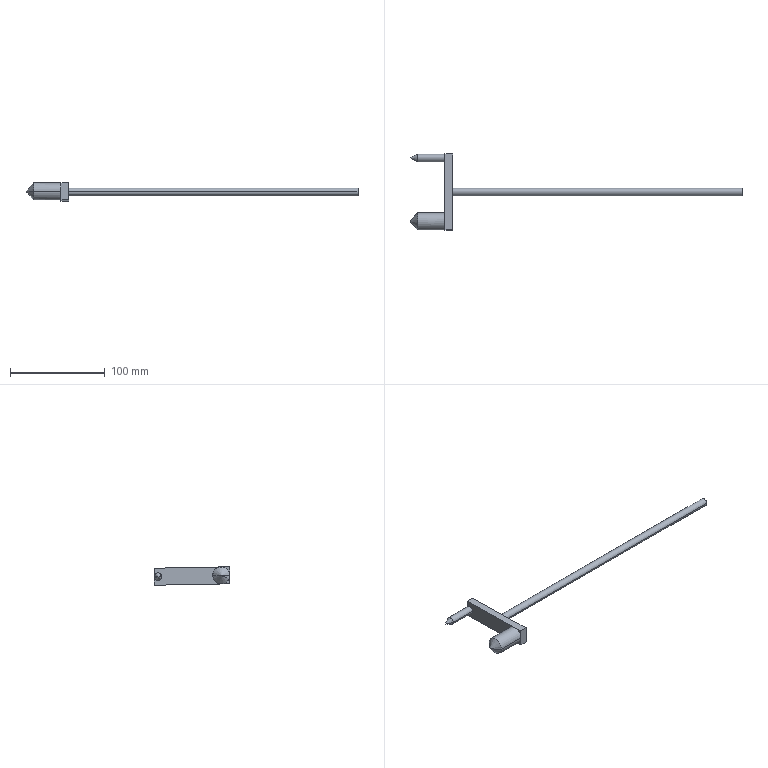Component | SolidWorks | RockerArm-1 | 1 solid | 19 faces | box 351 x 80.32 x 19.49 mm | volume 36551 mm3 | plane 9 | cylinder 6 | cone 4 | commonest cylinder face diameters 8 x4 18 x2
build123d program:
from build123d import *

# Parameters (mm, degrees)
SKETCH1_R           = 4
BOSS_EXTRUDE1_DEPTH = 306
SKETCH2_W           = 80
SKETCH2_H           = 18
BOSS_EXTRUDE2_DEPTH = 8
SKETCH4_R           = 9
SKETCH4_R_2         = 4
BOSS_EXTRUDE3_DEPTH = 37
CUT_EXTRUDE1_START  = -8
SKETCH6_R           = 9
CUT_EXTRUDE1_DEPTH  = 8
CUT_EXTRUDE2_START  = -8
SKETCH7_R           = 4
CUT_EXTRUDE2_DEPTH  = 8


with BuildPart() as part:
    # Sketch1 → Boss-Extrude1 (new body)
    with BuildSketch(Plane(origin=(0, 0, 0), x_dir=(0, 0, -1), z_dir=(1, 0, 0))):
        Circle(SKETCH1_R)
    extrude(amount=BOSS_EXTRUDE1_DEPTH)

    # Sketch2 → Boss-Extrude2 (add)
    with BuildSketch(Plane(origin=(306, 0, 0), x_dir=(0, 0, -1), z_dir=(1, 0, 0))):
        Rectangle(SKETCH2_W, SKETCH2_H)
    extrude(amount=BOSS_EXTRUDE2_DEPTH)

    # Sketch4 → Boss-Extrude3 (add)
    with BuildSketch(Plane(origin=(314, 0, 0), x_dir=(0, 0, -1), z_dir=(1, 0, 0))):
        with Locations(Location((-31, 0, 0), (0, 0, 180))):
            Circle(SKETCH4_R)
        with Locations((36, 0)):
            Circle(SKETCH4_R_2)
    extrude(amount=BOSS_EXTRUDE3_DEPTH)

    # Sketch6 → Cut-Extrude1 (cut)
    with BuildSketch(Plane(origin=(351, 0, 0), x_dir=(0, 0, -1), z_dir=(1, 0, 0)).offset(CUT_EXTRUDE1_START)):
        with Locations(Location((-31, 0, 0), (0, 0, 180))):
            Circle(SKETCH6_R)
    extrude(amount=CUT_EXTRUDE1_DEPTH, mode=Mode.SUBTRACT)

    # Sketch5 → Revolve1 (revolve)
    with BuildSketch(Plane(origin=(0, 0, 0), x_dir=(1, 0, 0), z_dir=(0, 1, 0)), mode=Mode.PRIVATE) as revolve1_sk:
        Polygon((351, -31), (343, -31), (343, -22), align=None)
    revolve(revolve1_sk.sketch.rotate(Axis((351, 0, 31), (-1, 0, 0)), 180), axis=Axis((351, 0, 31), (-1, 0, 0)))

    # Sketch7 → Cut-Extrude2 (cut)
    with BuildSketch(Plane(origin=(351, 0, 0), x_dir=(0, 0, -1), z_dir=(1, 0, 0)).offset(CUT_EXTRUDE2_START)):
        with Locations((36, 0)):
            Circle(SKETCH7_R)
    extrude(amount=CUT_EXTRUDE2_DEPTH, mode=Mode.SUBTRACT)

    # Sketch8 → Revolve2 (revolve)
    with BuildSketch(Plane(origin=(0, 0, 0), x_dir=(1, 0, 0), z_dir=(0, 1, 0)), mode=Mode.PRIVATE) as revolve2_sk:
        Polygon((343, 36), (351, 36), (343, 40), align=None)
    revolve(revolve2_sk.sketch.rotate(Axis((343, 0, -36), (1, 0, 0)), 180), axis=Axis((343, 0, -36), (1, 0, 0)))


solid = part.part

# Placed as in the assembly
solid = solid.moved(Location((890.528, 15.81, -277), (88.932, 0, -180)))
STEP:
#1=COLOUR_RGB('',0.7922,0.8196,0.9333);
#2=FILL_AREA_STYLE_COLOUR('',#1);
#3=FILL_AREA_STYLE('',(#2));
#4=SURFACE_STYLE_FILL_AREA(#3);
#5=SURFACE_SIDE_STYLE('',(#4));
#6=SURFACE_STYLE_USAGE(.BOTH.,#5);
#7=PRESENTATION_STYLE_ASSIGNMENT((#6));
#8=CARTESIAN_POINT('',(21.241,2.04,-10.932));
#9=VERTEX_POINT('',#8);
#10=CARTESIAN_POINT('',(21.556,1.882,-10.929));
#11=VERTEX_POINT('',#10);
#12=CARTESIAN_POINT('',(21.241,2.04,-10.932));
#13=DIRECTION('',(0.8944,-0.4471,0.008333));
#14=VECTOR('',#13,39.37);
#15=LINE('',#12,#14);
#16=EDGE_CURVE('',#9,#11,#15,.T.);
#17=ORIENTED_EDGE('',*,*,#16,.F.);
#18=CARTESIAN_POINT('',(21.556,2.197,-10.935));
#19=VERTEX_POINT('',#18);
#20=CARTESIAN_POINT('',(21.241,2.04,-10.932));
#21=DIRECTION('',(0.8944,0.4471,-0.008333));
#22=VECTOR('',#21,39.37);
#23=LINE('',#20,#22);
#24=EDGE_CURVE('',#9,#19,#23,.T.);
#25=ORIENTED_EDGE('',*,*,#24,.T.);
#26=CARTESIAN_POINT('',(21.556,2.04,-10.932));
#27=DIRECTION('',(-1.,-0.,-0.));
#28=DIRECTION('',(0.,0.9998,-0.01863));
#29=AXIS2_PLACEMENT_3D('',#26,#27,#28);
#30=CIRCLE('',#29,0.1575);
#31=EDGE_CURVE('',#19,#11,#30,.T.);
#32=ORIENTED_EDGE('',*,*,#31,.T.);
#33=EDGE_LOOP('',(#17,#25,#32));
#34=FACE_OUTER_BOUND('',#33,.T.);
#35=CARTESIAN_POINT('',(60.611,2.04,-10.932));
#36=DIRECTION('',(1.,0.,0.));
#37=DIRECTION('',(0.,-0.9998,0.01863));
#38=AXIS2_PLACEMENT_3D('',#35,#36,#37);
#39=CONICAL_SURFACE('',#38,19.685,0.4636);
#40=ADVANCED_FACE('',(#34),#39,.T.);
#41=CARTESIAN_POINT('',(21.241,-0.5978,-10.883));
#42=VERTEX_POINT('',#41);
#43=CARTESIAN_POINT('',(21.556,-0.9521,-10.876));
#44=VERTEX_POINT('',#43);
#45=CARTESIAN_POINT('',(21.241,-0.5978,-10.883));
#46=DIRECTION('',(0.6644,-0.7473,0.01393));
#47=VECTOR('',#46,39.37);
#48=LINE('',#45,#47);
#49=EDGE_CURVE('',#42,#44,#48,.T.);
#50=ORIENTED_EDGE('',*,*,#49,.F.);
#51=CARTESIAN_POINT('',(21.556,-0.2435,-10.889));
#52=VERTEX_POINT('',#51);
#53=CARTESIAN_POINT('',(21.241,-0.5978,-10.883));
#54=DIRECTION('',(0.6644,0.7473,-0.01393));
#55=VECTOR('',#54,39.37);
#56=LINE('',#53,#55);
#57=EDGE_CURVE('',#42,#52,#56,.T.);
#58=ORIENTED_EDGE('',*,*,#57,.T.);
#59=CARTESIAN_POINT('',(21.556,-0.5978,-10.883));
#60=DIRECTION('',(-1.,-0.,-0.));
#61=DIRECTION('',(0.,0.9998,-0.01863));
#62=AXIS2_PLACEMENT_3D('',#59,#60,#61);
#63=CIRCLE('',#62,0.3543);
#64=EDGE_CURVE('',#52,#44,#63,.T.);
#65=ORIENTED_EDGE('',*,*,#64,.T.);
#66=EDGE_LOOP('',(#50,#58,#65));
#67=FACE_OUTER_BOUND('',#66,.T.);
#68=CARTESIAN_POINT('',(60.611,-0.5978,-10.883));
#69=DIRECTION('',(1.,0.,0.));
#70=DIRECTION('',(0.,-0.9998,0.01863));
#71=AXIS2_PLACEMENT_3D('',#68,#69,#70);
#72=CONICAL_SURFACE('',#71,44.291,0.8442);
#73=ADVANCED_FACE('',(#67),#72,.T.);
#74=CARTESIAN_POINT('',(23.013,0.7799,-10.908));
#75=VERTEX_POINT('',#74);
#76=CARTESIAN_POINT('',(23.013,0.465,-10.903));
#77=VERTEX_POINT('',#76);
#78=CARTESIAN_POINT('',(23.013,0.6225,-10.906));
#79=DIRECTION('',(-1.,-0.,-0.));
#80=DIRECTION('',(0.,0.9998,-0.01863));
#81=AXIS2_PLACEMENT_3D('',#78,#79,#80);
#82=CIRCLE('',#81,0.1575);
#83=EDGE_CURVE('',#75,#77,#82,.T.);
#84=ORIENTED_EDGE('',*,*,#83,.F.);
#85=CARTESIAN_POINT('',(35.06,0.7799,-10.908));
#86=VERTEX_POINT('',#85);
#87=CARTESIAN_POINT('',(23.013,0.7799,-10.908));
#88=DIRECTION('',(1.,0.,0.));
#89=VECTOR('',#88,39.37);
#90=LINE('',#87,#89);
#91=EDGE_CURVE('',#75,#86,#90,.T.);
#92=ORIENTED_EDGE('',*,*,#91,.T.);
#93=CARTESIAN_POINT('',(35.06,0.465,-10.903));
#94=VERTEX_POINT('',#93);
#95=CARTESIAN_POINT('',(35.06,0.6225,-10.906));
#96=DIRECTION('',(-1.,-0.,-0.));
#97=DIRECTION('',(0.,0.9998,-0.01863));
#98=AXIS2_PLACEMENT_3D('',#95,#96,#97);
#99=CIRCLE('',#98,0.1575);
#100=EDGE_CURVE('',#86,#94,#99,.T.);
#101=ORIENTED_EDGE('',*,*,#100,.T.);
#102=CARTESIAN_POINT('',(23.013,0.465,-10.903));
#103=DIRECTION('',(1.,0.,0.));
#104=VECTOR('',#103,39.37);
#105=LINE('',#102,#104);
#106=EDGE_CURVE('',#77,#94,#105,.T.);
#107=ORIENTED_EDGE('',*,*,#106,.F.);
#108=EDGE_LOOP('',(#84,#92,#101,#107));
#109=FACE_OUTER_BOUND('',#108,.T.);
#110=CARTESIAN_POINT('',(23.013,0.6225,-10.906));
#111=DIRECTION('',(1.,0.,0.));
#112=DIRECTION('',(0.,-0.9998,0.01863));
#113=AXIS2_PLACEMENT_3D('',#110,#111,#112);
#114=CYLINDRICAL_SURFACE('',#113,0.1575);
#115=ADVANCED_FACE('',(#109),#114,.T.);
#116=ORIENTED_EDGE('',*,*,#64,.F.);
#117=CARTESIAN_POINT('',(22.698,-0.2435,-10.889));
#118=VERTEX_POINT('',#117);
#119=CARTESIAN_POINT('',(21.241,-0.2435,-10.889));
#120=DIRECTION('',(1.,0.,0.));
#121=VECTOR('',#120,39.37);
#122=LINE('',#119,#121);
#123=EDGE_CURVE('',#52,#118,#122,.T.);
#124=ORIENTED_EDGE('',*,*,#123,.T.);
#125=CARTESIAN_POINT('',(22.698,-0.6044,-11.237));
#126=VERTEX_POINT('',#125);
#127=CARTESIAN_POINT('',(22.698,-0.5978,-10.883));
#128=DIRECTION('',(-1.,-0.,-0.));
#129=DIRECTION('',(0.,0.9998,-0.01863));
#130=AXIS2_PLACEMENT_3D('',#127,#128,#129);
#131=CIRCLE('',#130,0.3543);
#132=EDGE_CURVE('',#118,#126,#131,.T.);
#133=ORIENTED_EDGE('',*,*,#132,.T.);
#134=CARTESIAN_POINT('',(22.698,-0.9521,-10.876));
#135=VERTEX_POINT('',#134);
#136=CARTESIAN_POINT('',(22.698,-0.5978,-10.883));
#137=DIRECTION('',(-1.,-0.,-0.));
#138=DIRECTION('',(0.,0.9998,-0.01863));
#139=AXIS2_PLACEMENT_3D('',#136,#137,#138);
#140=CIRCLE('',#139,0.3543);
#141=EDGE_CURVE('',#126,#135,#140,.T.);
#142=ORIENTED_EDGE('',*,*,#141,.T.);
#143=CARTESIAN_POINT('',(21.241,-0.9521,-10.876));
#144=DIRECTION('',(1.,0.,0.));
#145=VECTOR('',#144,39.37);
#146=LINE('',#143,#145);
#147=EDGE_CURVE('',#44,#135,#146,.T.);
#148=ORIENTED_EDGE('',*,*,#147,.F.);
#149=EDGE_LOOP('',(#116,#124,#133,#142,#148));
#150=FACE_OUTER_BOUND('',#149,.T.);
#151=CARTESIAN_POINT('',(21.241,-0.5978,-10.883));
#152=DIRECTION('',(1.,0.,0.));
#153=DIRECTION('',(0.,-0.9998,0.01863));
#154=AXIS2_PLACEMENT_3D('',#151,#152,#153);
#155=CYLINDRICAL_SURFACE('',#154,0.3543);
#156=ADVANCED_FACE('',(#150),#155,.T.);
#157=ORIENTED_EDGE('',*,*,#31,.F.);
#158=CARTESIAN_POINT('',(22.698,2.197,-10.935));
#159=VERTEX_POINT('',#158);
#160=CARTESIAN_POINT('',(21.241,2.197,-10.935));
#161=DIRECTION('',(1.,0.,0.));
#162=VECTOR('',#161,39.37);
#163=LINE('',#160,#162);
#164=EDGE_CURVE('',#19,#159,#163,.T.);
#165=ORIENTED_EDGE('',*,*,#164,.T.);
#166=CARTESIAN_POINT('',(22.698,1.882,-10.929));
#167=VERTEX_POINT('',#166);
#168=CARTESIAN_POINT('',(22.698,2.04,-10.932));
#169=DIRECTION('',(-1.,-0.,-0.));
#170=DIRECTION('',(0.,0.9998,-0.01863));
#171=AXIS2_PLACEMENT_3D('',#168,#169,#170);
#172=CIRCLE('',#171,0.1575);
#173=EDGE_CURVE('',#159,#167,#172,.T.);
#174=ORIENTED_EDGE('',*,*,#173,.T.);
#175=CARTESIAN_POINT('',(21.241,1.882,-10.929));
#176=DIRECTION('',(1.,0.,0.));
#177=VECTOR('',#176,39.37);
#178=LINE('',#175,#177);
#179=EDGE_CURVE('',#11,#167,#178,.T.);
#180=ORIENTED_EDGE('',*,*,#179,.F.);
#181=EDGE_LOOP('',(#157,#165,#174,#180));
#182=FACE_OUTER_BOUND('',#181,.T.);
#183=CARTESIAN_POINT('',(21.241,2.04,-10.932));
#184=DIRECTION('',(1.,0.,0.));
#185=DIRECTION('',(0.,-0.9998,0.01863));
#186=AXIS2_PLACEMENT_3D('',#183,#184,#185);
#187=CYLINDRICAL_SURFACE('',#186,0.1575);
#188=ADVANCED_FACE('',(#182),#187,.T.);
#189=ORIENTED_EDGE('',*,*,#164,.F.);
#190=CARTESIAN_POINT('',(21.556,2.04,-10.932));
#191=DIRECTION('',(-1.,-0.,-0.));
#192=DIRECTION('',(0.,0.9998,-0.01863));
#193=AXIS2_PLACEMENT_3D('',#190,#191,#192);
#194=CIRCLE('',#193,0.1575);
#195=EDGE_CURVE('',#11,#19,#194,.T.);
#196=ORIENTED_EDGE('',*,*,#195,.F.);
#197=ORIENTED_EDGE('',*,*,#179,.T.);
#198=CARTESIAN_POINT('',(22.698,2.04,-10.932));
#199=DIRECTION('',(-1.,-0.,-0.));
#200=DIRECTION('',(0.,0.9998,-0.01863));
#201=AXIS2_PLACEMENT_3D('',#198,#199,#200);
#202=CIRCLE('',#201,0.1575);
#203=EDGE_CURVE('',#167,#159,#202,.T.);
#204=ORIENTED_EDGE('',*,*,#203,.T.);
#205=EDGE_LOOP('',(#189,#196,#197,#204));
#206=FACE_OUTER_BOUND('',#205,.T.);
#207=CARTESIAN_POINT('',(21.241,2.04,-10.932));
#208=DIRECTION('',(1.,0.,0.));
#209=DIRECTION('',(0.,-0.9998,0.01863));
#210=AXIS2_PLACEMENT_3D('',#207,#208,#209);
#211=CYLINDRICAL_SURFACE('',#210,0.1575);
#212=ADVANCED_FACE('',(#206),#211,.T.);
#213=ORIENTED_EDGE('',*,*,#123,.F.);
#214=CARTESIAN_POINT('',(21.556,-0.5978,-10.883));
#215=DIRECTION('',(-1.,-0.,-0.));
#216=DIRECTION('',(0.,0.9998,-0.01863));
#217=AXIS2_PLACEMENT_3D('',#214,#215,#216);
#218=CIRCLE('',#217,0.3543);
#219=EDGE_CURVE('',#44,#52,#218,.T.);
#220=ORIENTED_EDGE('',*,*,#219,.F.);
#221=ORIENTED_EDGE('',*,*,#147,.T.);
#222=CARTESIAN_POINT('',(22.698,-0.5912,-10.529));
#223=VERTEX_POINT('',#222);
#224=CARTESIAN_POINT('',(22.698,-0.5978,-10.883));
#225=DIRECTION('',(-1.,-0.,-0.));
#226=DIRECTION('',(0.,0.9998,-0.01863));
#227=AXIS2_PLACEMENT_3D('',#224,#225,#226);
#228=CIRCLE('',#227,0.3543);
#229=EDGE_CURVE('',#135,#223,#228,.T.);
#230=ORIENTED_EDGE('',*,*,#229,.T.);
#231=CARTESIAN_POINT('',(22.698,-0.5978,-10.883));
#232=DIRECTION('',(-1.,-0.,-0.));
#233=DIRECTION('',(0.,0.9998,-0.01863));
#234=AXIS2_PLACEMENT_3D('',#231,#232,#233);
#235=CIRCLE('',#234,0.3543);
#236=EDGE_CURVE('',#223,#118,#235,.T.);
#237=ORIENTED_EDGE('',*,*,#236,.T.);
#238=EDGE_LOOP('',(#213,#220,#221,#230,#237));
#239=FACE_OUTER_BOUND('',#238,.T.);
#240=CARTESIAN_POINT('',(21.241,-0.5978,-10.883));
#241=DIRECTION('',(1.,0.,0.));
#242=DIRECTION('',(0.,-0.9998,0.01863));
#243=AXIS2_PLACEMENT_3D('',#240,#241,#242);
#244=CYLINDRICAL_SURFACE('',#243,0.3543);
#245=ADVANCED_FACE('',(#239),#244,.T.);
#246=CARTESIAN_POINT('',(22.698,2.204,-10.581));
#247=VERTEX_POINT('',#246);
#248=CARTESIAN_POINT('',(22.698,2.19,-11.289));
#249=DIRECTION('',(0.,-0.01863,-0.9998));
#250=VECTOR('',#249,39.37);
#251=LINE('',#248,#250);
#252=EDGE_CURVE('',#247,#159,#251,.T.);
#253=ORIENTED_EDGE('',*,*,#252,.T.);
#254=ORIENTED_EDGE('',*,*,#203,.F.);
#255=ORIENTED_EDGE('',*,*,#173,.F.);
#256=CARTESIAN_POINT('',(22.698,2.19,-11.289));
#257=VERTEX_POINT('',#256);
#258=CARTESIAN_POINT('',(22.698,2.19,-11.289));
#259=DIRECTION('',(0.,-0.01863,-0.9998));
#260=VECTOR('',#259,39.37);
#261=LINE('',#258,#260);
#262=EDGE_CURVE('',#159,#257,#261,.T.);
#263=ORIENTED_EDGE('',*,*,#262,.T.);
#264=CARTESIAN_POINT('',(22.698,2.19,-11.289));
#265=DIRECTION('',(0.,-0.9998,0.01863));
#266=VECTOR('',#265,39.37);
#267=LINE('',#264,#266);
#268=EDGE_CURVE('',#257,#126,#267,.T.);
#269=ORIENTED_EDGE('',*,*,#268,.T.);
#270=ORIENTED_EDGE('',*,*,#132,.F.);
#271=ORIENTED_EDGE('',*,*,#236,.F.);
#272=CARTESIAN_POINT('',(22.698,2.204,-10.581));
#273=DIRECTION('',(-0.,0.9998,-0.01863));
#274=VECTOR('',#273,39.37);
#275=LINE('',#272,#274);
#276=EDGE_CURVE('',#223,#247,#275,.T.);
#277=ORIENTED_EDGE('',*,*,#276,.T.);
#278=EDGE_LOOP('',(#253,#254,#255,#263,#269,#270,#271,#277));
#279=FACE_OUTER_BOUND('',#278,.T.);
#280=CARTESIAN_POINT('',(22.698,0.6225,-10.906));
#281=DIRECTION('',(1.,0.,0.));
#282=DIRECTION('',(0.,-0.9998,0.01863));
#283=AXIS2_PLACEMENT_3D('',#280,#281,#282);
#284=PLANE('',#283);
#285=ADVANCED_FACE('',(#279),#284,.F.);
#286=ORIENTED_EDGE('',*,*,#141,.F.);
#287=CARTESIAN_POINT('',(22.698,-0.9587,-11.23));
#288=VERTEX_POINT('',#287);
#289=CARTESIAN_POINT('',(22.698,2.19,-11.289));
#290=DIRECTION('',(0.,-0.9998,0.01863));
#291=VECTOR('',#290,39.37);
#292=LINE('',#289,#291);
#293=EDGE_CURVE('',#126,#288,#292,.T.);
#294=ORIENTED_EDGE('',*,*,#293,.T.);
#295=CARTESIAN_POINT('',(22.698,-0.9587,-11.23));
#296=DIRECTION('',(-0.,0.01863,0.9998));
#297=VECTOR('',#296,39.37);
#298=LINE('',#295,#297);
#299=EDGE_CURVE('',#288,#135,#298,.T.);
#300=ORIENTED_EDGE('',*,*,#299,.T.);
#301=EDGE_LOOP('',(#286,#294,#300));
#302=FACE_OUTER_BOUND('',#301,.T.);
#303=CARTESIAN_POINT('',(22.698,0.6225,-10.906));
#304=DIRECTION('',(1.,0.,0.));
#305=DIRECTION('',(0.,-0.9998,0.01863));
#306=AXIS2_PLACEMENT_3D('',#303,#304,#305);
#307=PLANE('',#306);
#308=ADVANCED_FACE('',(#302),#307,.F.);
#309=ORIENTED_EDGE('',*,*,#229,.F.);
#310=CARTESIAN_POINT('',(22.698,-0.9455,-10.522));
#311=VERTEX_POINT('',#310);
#312=CARTESIAN_POINT('',(22.698,-0.9587,-11.23));
#313=DIRECTION('',(-0.,0.01863,0.9998));
#314=VECTOR('',#313,39.37);
#315=LINE('',#312,#314);
#316=EDGE_CURVE('',#135,#311,#315,.T.);
#317=ORIENTED_EDGE('',*,*,#316,.T.);
#318=CARTESIAN_POINT('',(22.698,2.204,-10.581));
#319=DIRECTION('',(-0.,0.9998,-0.01863));
#320=VECTOR('',#319,39.37);
#321=LINE('',#318,#320);
#322=EDGE_CURVE('',#311,#223,#321,.T.);
#323=ORIENTED_EDGE('',*,*,#322,.T.);
#324=EDGE_LOOP('',(#309,#317,#323));
#325=FACE_OUTER_BOUND('',#324,.T.);
#326=CARTESIAN_POINT('',(22.698,0.6225,-10.906));
#327=DIRECTION('',(1.,0.,0.));
#328=DIRECTION('',(0.,-0.9998,0.01863));
#329=AXIS2_PLACEMENT_3D('',#326,#327,#328);
#330=PLANE('',#329);
#331=ADVANCED_FACE('',(#325),#330,.F.);
#332=ORIENTED_EDGE('',*,*,#91,.F.);
#333=CARTESIAN_POINT('',(23.013,0.6225,-10.906));
#334=DIRECTION('',(-1.,-0.,-0.));
#335=DIRECTION('',(0.,0.9998,-0.01863));
#336=AXIS2_PLACEMENT_3D('',#333,#334,#335);
#337=CIRCLE('',#336,0.1575);
#338=EDGE_CURVE('',#77,#75,#337,.T.);
#339=ORIENTED_EDGE('',*,*,#338,.F.);
#340=ORIENTED_EDGE('',*,*,#106,.T.);
#341=CARTESIAN_POINT('',(35.06,0.6225,-10.906));
#342=DIRECTION('',(-1.,-0.,-0.));
#343=DIRECTION('',(0.,0.9998,-0.01863));
#344=AXIS2_PLACEMENT_3D('',#341,#342,#343);
#345=CIRCLE('',#344,0.1575);
#346=EDGE_CURVE('',#94,#86,#345,.T.);
#347=ORIENTED_EDGE('',*,*,#346,.T.);
#348=EDGE_LOOP('',(#332,#339,#340,#347));
#349=FACE_OUTER_BOUND('',#348,.T.);
#350=CARTESIAN_POINT('',(23.013,0.6225,-10.906));
#351=DIRECTION('',(1.,0.,0.));
#352=DIRECTION('',(0.,-0.9998,0.01863));
#353=AXIS2_PLACEMENT_3D('',#350,#351,#352);
#354=CYLINDRICAL_SURFACE('',#353,0.1575);
#355=ADVANCED_FACE('',(#349),#354,.T.);
#356=ORIENTED_EDGE('',*,*,#346,.F.);
#357=ORIENTED_EDGE('',*,*,#100,.F.);
#358=EDGE_LOOP('',(#356,#357));
#359=FACE_OUTER_BOUND('',#358,.T.);
#360=CARTESIAN_POINT('',(35.06,0.6225,-10.906));
#361=DIRECTION('',(-1.,-0.,-0.));
#362=DIRECTION('',(-0.,0.9998,-0.01863));
#363=AXIS2_PLACEMENT_3D('',#360,#361,#362);
#364=PLANE('',#363);
#365=ADVANCED_FACE('',(#359),#364,.F.);
#366=CARTESIAN_POINT('',(23.013,-0.9587,-11.23));
#367=VERTEX_POINT('',#366);
#368=CARTESIAN_POINT('',(23.013,-0.9455,-10.522));
#369=VERTEX_POINT('',#368);
#370=CARTESIAN_POINT('',(23.013,-0.9587,-11.23));
#371=DIRECTION('',(-0.,0.01863,0.9998));
#372=VECTOR('',#371,39.37);
#373=LINE('',#370,#372);
#374=EDGE_CURVE('',#367,#369,#373,.T.);
#375=ORIENTED_EDGE('',*,*,#374,.F.);
#376=CARTESIAN_POINT('',(23.013,2.19,-11.289));
#377=VERTEX_POINT('',#376);
#378=CARTESIAN_POINT('',(23.013,2.19,-11.289));
#379=DIRECTION('',(0.,-0.9998,0.01863));
#380=VECTOR('',#379,39.37);
#381=LINE('',#378,#380);
#382=EDGE_CURVE('',#377,#367,#381,.T.);
#383=ORIENTED_EDGE('',*,*,#382,.F.);
#384=CARTESIAN_POINT('',(23.013,2.204,-10.581));
#385=VERTEX_POINT('',#384);
#386=CARTESIAN_POINT('',(23.013,2.19,-11.289));
#387=DIRECTION('',(0.,-0.01863,-0.9998));
#388=VECTOR('',#387,39.37);
#389=LINE('',#386,#388);
#390=EDGE_CURVE('',#385,#377,#389,.T.);
#391=ORIENTED_EDGE('',*,*,#390,.F.);
#392=CARTESIAN_POINT('',(23.013,2.204,-10.581));
#393=DIRECTION('',(-0.,0.9998,-0.01863));
#394=VECTOR('',#393,39.37);
#395=LINE('',#392,#394);
#396=EDGE_CURVE('',#369,#385,#395,.T.);
#397=ORIENTED_EDGE('',*,*,#396,.F.);
#398=EDGE_LOOP('',(#375,#383,#391,#397));
#399=FACE_OUTER_BOUND('',#398,.T.);
#400=ORIENTED_EDGE('',*,*,#338,.T.);
#401=ORIENTED_EDGE('',*,*,#83,.T.);
#402=EDGE_LOOP('',(#400,#401));
#403=FACE_BOUND('',#402,.T.);
#404=CARTESIAN_POINT('',(23.013,0.6225,-10.906));
#405=DIRECTION('',(1.,0.,0.));
#406=DIRECTION('',(0.,-0.9998,0.01863));
#407=AXIS2_PLACEMENT_3D('',#404,#405,#406);
#408=PLANE('',#407);
#409=ADVANCED_FACE('',(#399,#403),#408,.T.);
#410=ORIENTED_EDGE('',*,*,#374,.T.);
#411=CARTESIAN_POINT('',(22.698,-0.9455,-10.522));
#412=DIRECTION('',(1.,0.,0.));
#413=VECTOR('',#412,39.37);
#414=LINE('',#411,#413);
#415=EDGE_CURVE('',#311,#369,#414,.T.);
#416=ORIENTED_EDGE('',*,*,#415,.F.);
#417=ORIENTED_EDGE('',*,*,#316,.F.);
#418=ORIENTED_EDGE('',*,*,#299,.F.);
#419=CARTESIAN_POINT('',(22.698,-0.9587,-11.23));
#420=DIRECTION('',(1.,0.,0.));
#421=VECTOR('',#420,39.37);
#422=LINE('',#419,#421);
#423=EDGE_CURVE('',#288,#367,#422,.T.);
#424=ORIENTED_EDGE('',*,*,#423,.T.);
#425=EDGE_LOOP('',(#410,#416,#417,#418,#424));
#426=FACE_OUTER_BOUND('',#425,.T.);
#427=CARTESIAN_POINT('',(22.698,-0.9587,-11.23));
#428=DIRECTION('',(-0.,0.9998,-0.01863));
#429=DIRECTION('',(1.,0.,0.));
#430=AXIS2_PLACEMENT_3D('',#427,#428,#429);
#431=PLANE('',#430);
#432=ADVANCED_FACE('',(#426),#431,.F.);
#433=ORIENTED_EDGE('',*,*,#396,.T.);
#434=CARTESIAN_POINT('',(22.698,2.204,-10.581));
#435=DIRECTION('',(1.,0.,0.));
#436=VECTOR('',#435,39.37);
#437=LINE('',#434,#436);
#438=EDGE_CURVE('',#247,#385,#437,.T.);
#439=ORIENTED_EDGE('',*,*,#438,.F.);
#440=ORIENTED_EDGE('',*,*,#276,.F.);
#441=ORIENTED_EDGE('',*,*,#322,.F.);
#442=ORIENTED_EDGE('',*,*,#415,.T.);
#443=EDGE_LOOP('',(#433,#439,#440,#441,#442));
#444=FACE_OUTER_BOUND('',#443,.T.);
#445=CARTESIAN_POINT('',(22.698,2.204,-10.581));
#446=DIRECTION('',(0.,-0.01863,-0.9998));
#447=DIRECTION('',(0.,-0.9998,0.01863));
#448=AXIS2_PLACEMENT_3D('',#445,#446,#447);
#449=PLANE('',#448);
#450=ADVANCED_FACE('',(#444),#449,.F.);
#451=ORIENTED_EDGE('',*,*,#390,.T.);
#452=CARTESIAN_POINT('',(22.698,2.19,-11.289));
#453=DIRECTION('',(1.,0.,0.));
#454=VECTOR('',#453,39.37);
#455=LINE('',#452,#454);
#456=EDGE_CURVE('',#257,#377,#455,.T.);
#457=ORIENTED_EDGE('',*,*,#456,.F.);
#458=ORIENTED_EDGE('',*,*,#262,.F.);
#459=ORIENTED_EDGE('',*,*,#252,.F.);
#460=ORIENTED_EDGE('',*,*,#438,.T.);
#461=EDGE_LOOP('',(#451,#457,#458,#459,#460));
#462=FACE_OUTER_BOUND('',#461,.T.);
#463=CARTESIAN_POINT('',(22.698,2.19,-11.289));
#464=DIRECTION('',(0.,-0.9998,0.01863));
#465=DIRECTION('',(-1.,-0.,-0.));
#466=AXIS2_PLACEMENT_3D('',#463,#464,#465);
#467=PLANE('',#466);
#468=ADVANCED_FACE('',(#462),#467,.F.);
#469=ORIENTED_EDGE('',*,*,#382,.T.);
#470=ORIENTED_EDGE('',*,*,#423,.F.);
#471=ORIENTED_EDGE('',*,*,#293,.F.);
#472=ORIENTED_EDGE('',*,*,#268,.F.);
#473=ORIENTED_EDGE('',*,*,#456,.T.);
#474=EDGE_LOOP('',(#469,#470,#471,#472,#473));
#475=FACE_OUTER_BOUND('',#474,.T.);
#476=CARTESIAN_POINT('',(22.698,2.19,-11.289));
#477=DIRECTION('',(-0.,0.01863,0.9998));
#478=DIRECTION('',(-0.,0.9998,-0.01863));
#479=AXIS2_PLACEMENT_3D('',#476,#477,#478);
#480=PLANE('',#479);
#481=ADVANCED_FACE('',(#475),#480,.F.);
#482=ORIENTED_EDGE('',*,*,#57,.F.);
#483=ORIENTED_EDGE('',*,*,#49,.T.);
#484=ORIENTED_EDGE('',*,*,#219,.T.);
#485=EDGE_LOOP('',(#482,#483,#484));
#486=FACE_OUTER_BOUND('',#485,.T.);
#487=CARTESIAN_POINT('',(60.611,-0.5978,-10.883));
#488=DIRECTION('',(1.,0.,0.));
#489=DIRECTION('',(0.,-0.9998,0.01863));
#490=AXIS2_PLACEMENT_3D('',#487,#488,#489);
#491=CONICAL_SURFACE('',#490,44.291,0.8442);
#492=ADVANCED_FACE('',(#486),#491,.T.);
#493=ORIENTED_EDGE('',*,*,#24,.F.);
#494=ORIENTED_EDGE('',*,*,#16,.T.);
#495=ORIENTED_EDGE('',*,*,#195,.T.);
#496=EDGE_LOOP('',(#493,#494,#495));
#497=FACE_OUTER_BOUND('',#496,.T.);
#498=CARTESIAN_POINT('',(60.611,2.04,-10.932));
#499=DIRECTION('',(1.,0.,0.));
#500=DIRECTION('',(0.,-0.9998,0.01863));
#501=AXIS2_PLACEMENT_3D('',#498,#499,#500);
#502=CONICAL_SURFACE('',#501,19.685,0.4636);
#503=ADVANCED_FACE('',(#497),#502,.T.);
#504=CLOSED_SHELL('',(#40,#73,#115,#156,#188,#212,#245,#285,#308,#331,#355,#365,#409,#432,#450,#468,#481,#492,#503));
#505=MANIFOLD_SOLID_BREP('',#504);
#506=STYLED_ITEM('',(#7),#505);
#507=(LENGTH_UNIT()NAMED_UNIT(*)SI_UNIT($,.METRE.));
#508=LENGTH_MEASURE_WITH_UNIT(LENGTH_MEASURE(0.0254),#507);
#509=DIMENSIONAL_EXPONENTS(1.,0.,0.,0.,0.,0.,0.);
#510=(CONVERSION_BASED_UNIT('',#508)LENGTH_UNIT()NAMED_UNIT(#509));
#511=UNCERTAINTY_MEASURE_WITH_UNIT(LENGTH_MEASURE(0.00001),#510,'','');
#512=(NAMED_UNIT(*)PLANE_ANGLE_UNIT()SI_UNIT($,.RADIAN.));
#513=(NAMED_UNIT(*)SI_UNIT($,.STERADIAN.)SOLID_ANGLE_UNIT());
#514=(GEOMETRIC_REPRESENTATION_CONTEXT(3)GLOBAL_UNCERTAINTY_ASSIGNED_CONTEXT((#511))GLOBAL_UNIT_ASSIGNED_CONTEXT((#510,#512,#513))REPRESENTATION_CONTEXT('',''));
#515=MECHANICAL_DESIGN_GEOMETRIC_PRESENTATION_REPRESENTATION('',(#506),#514);
#516=PRESENTATION_LAYER_ASSIGNMENT('','',(#506));
#517=CARTESIAN_POINT('',(0.,0.,0.));
#518=DIRECTION('',(0.,0.,1.));
#519=DIRECTION('',(1.,0.,0.));
#520=AXIS2_PLACEMENT_3D('',#517,#518,#519);
#521=(LENGTH_UNIT()NAMED_UNIT(*)SI_UNIT($,.METRE.));
#522=LENGTH_MEASURE_WITH_UNIT(LENGTH_MEASURE(0.0254),#521);
#523=DIMENSIONAL_EXPONENTS(1.,0.,0.,0.,0.,0.,0.);
#524=(CONVERSION_BASED_UNIT('',#522)LENGTH_UNIT()NAMED_UNIT(#523));
#525=UNCERTAINTY_MEASURE_WITH_UNIT(LENGTH_MEASURE(0.00001),#524,'','');
#526=(NAMED_UNIT(*)PLANE_ANGLE_UNIT()SI_UNIT($,.RADIAN.));
#527=(NAMED_UNIT(*)SI_UNIT($,.STERADIAN.)SOLID_ANGLE_UNIT());
#528=(GEOMETRIC_REPRESENTATION_CONTEXT(3)GLOBAL_UNCERTAINTY_ASSIGNED_CONTEXT((#525))GLOBAL_UNIT_ASSIGNED_CONTEXT((#524,#526,#527))REPRESENTATION_CONTEXT('',''));
#529=ADVANCED_BREP_SHAPE_REPRESENTATION('',(#505,#520),#528);